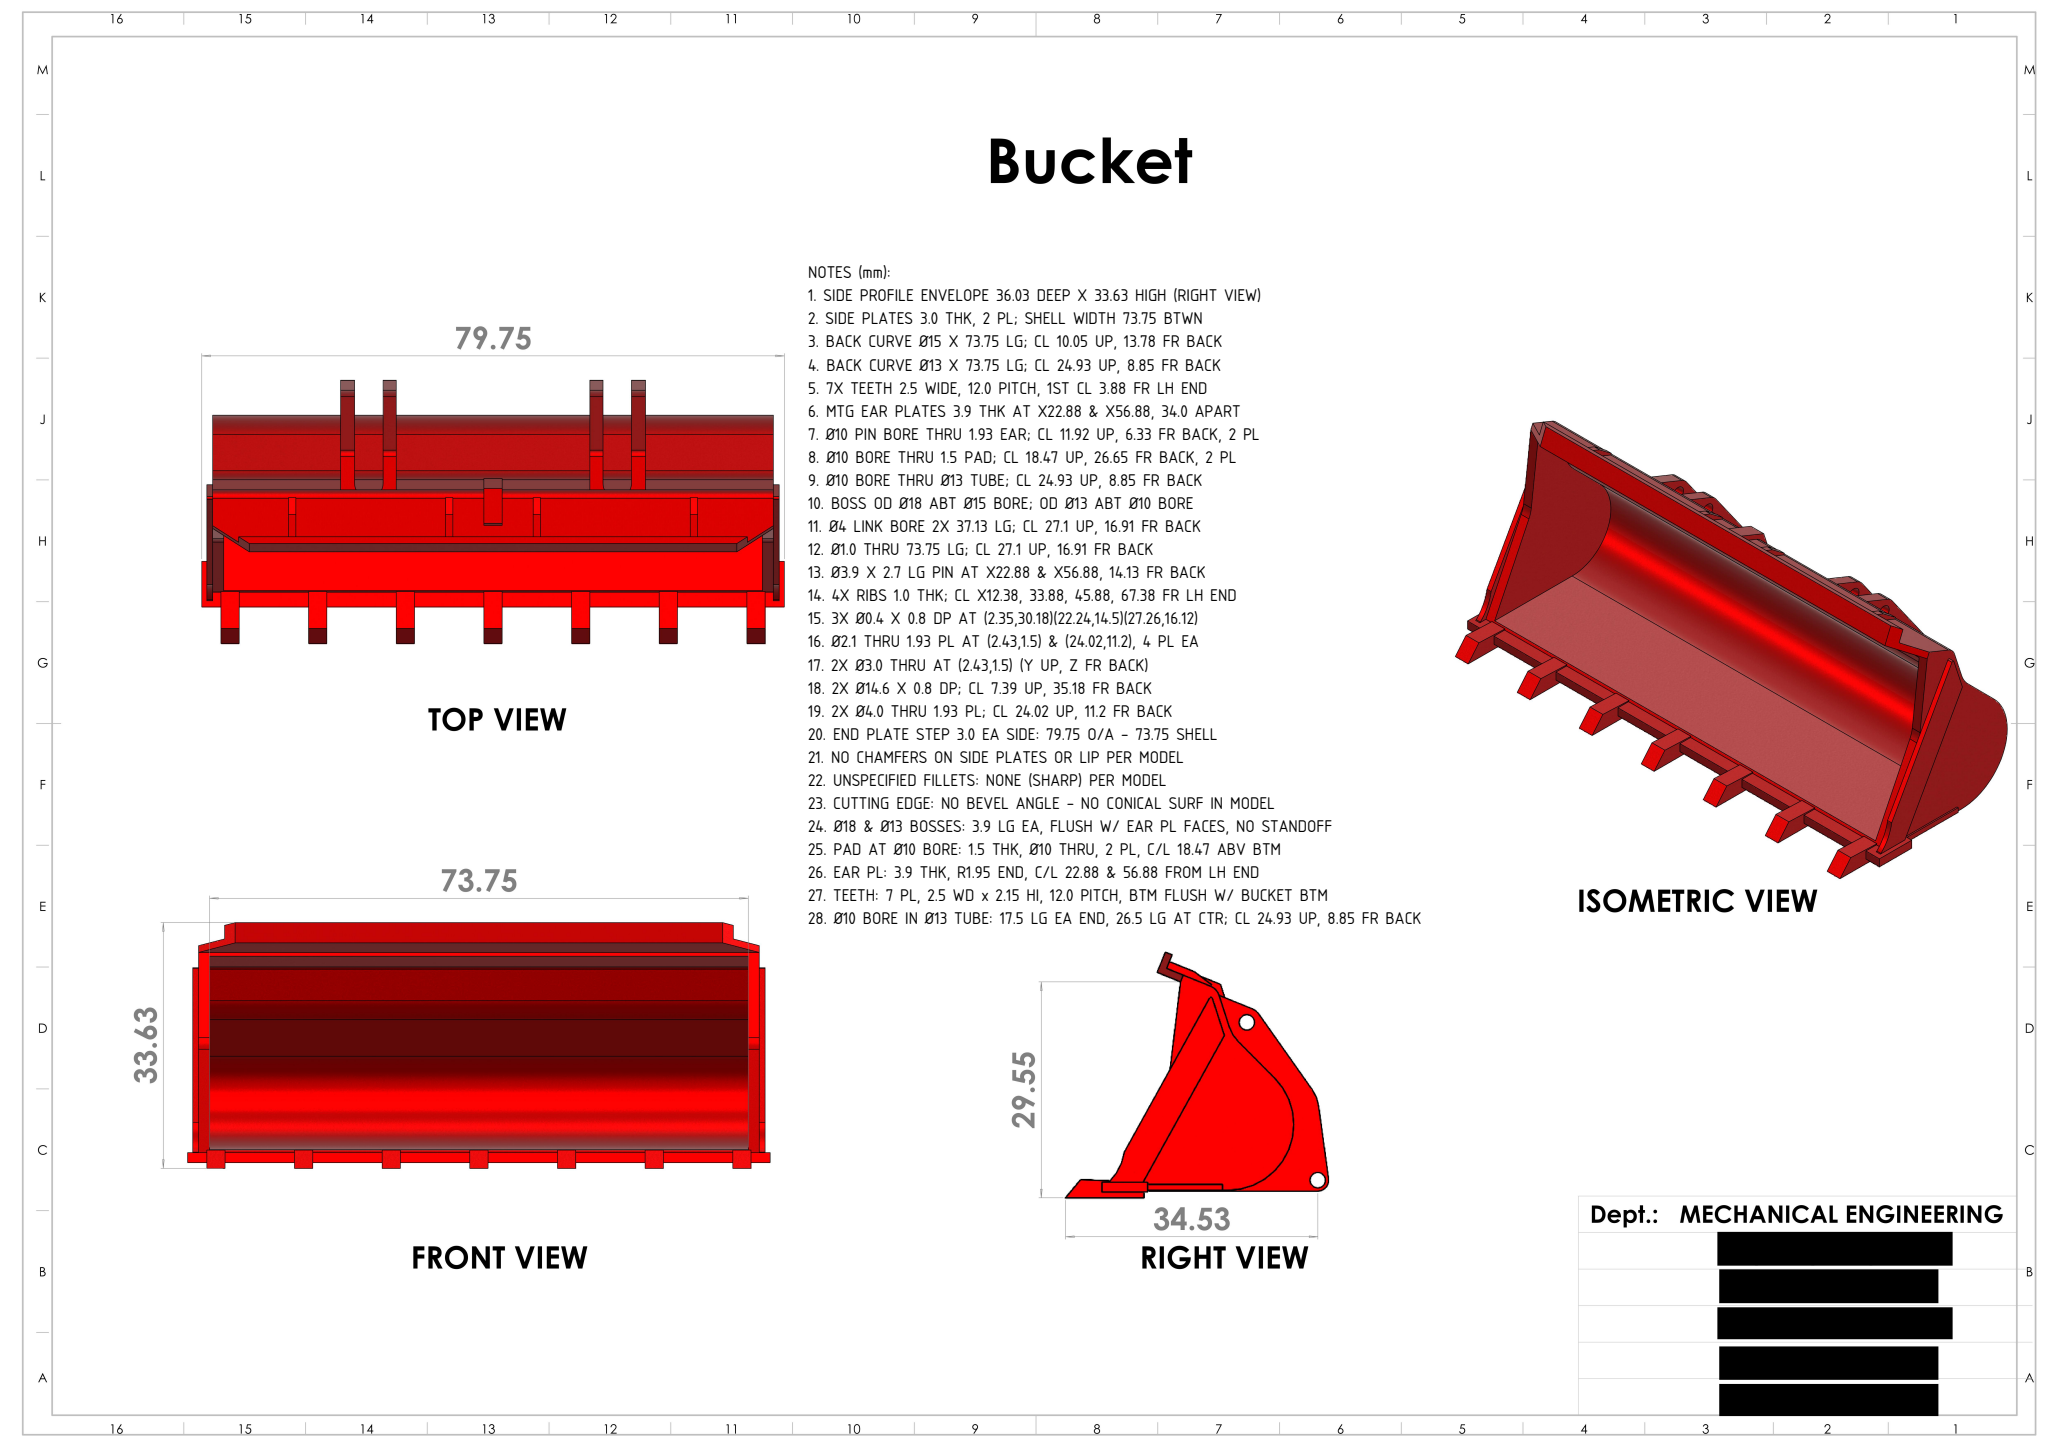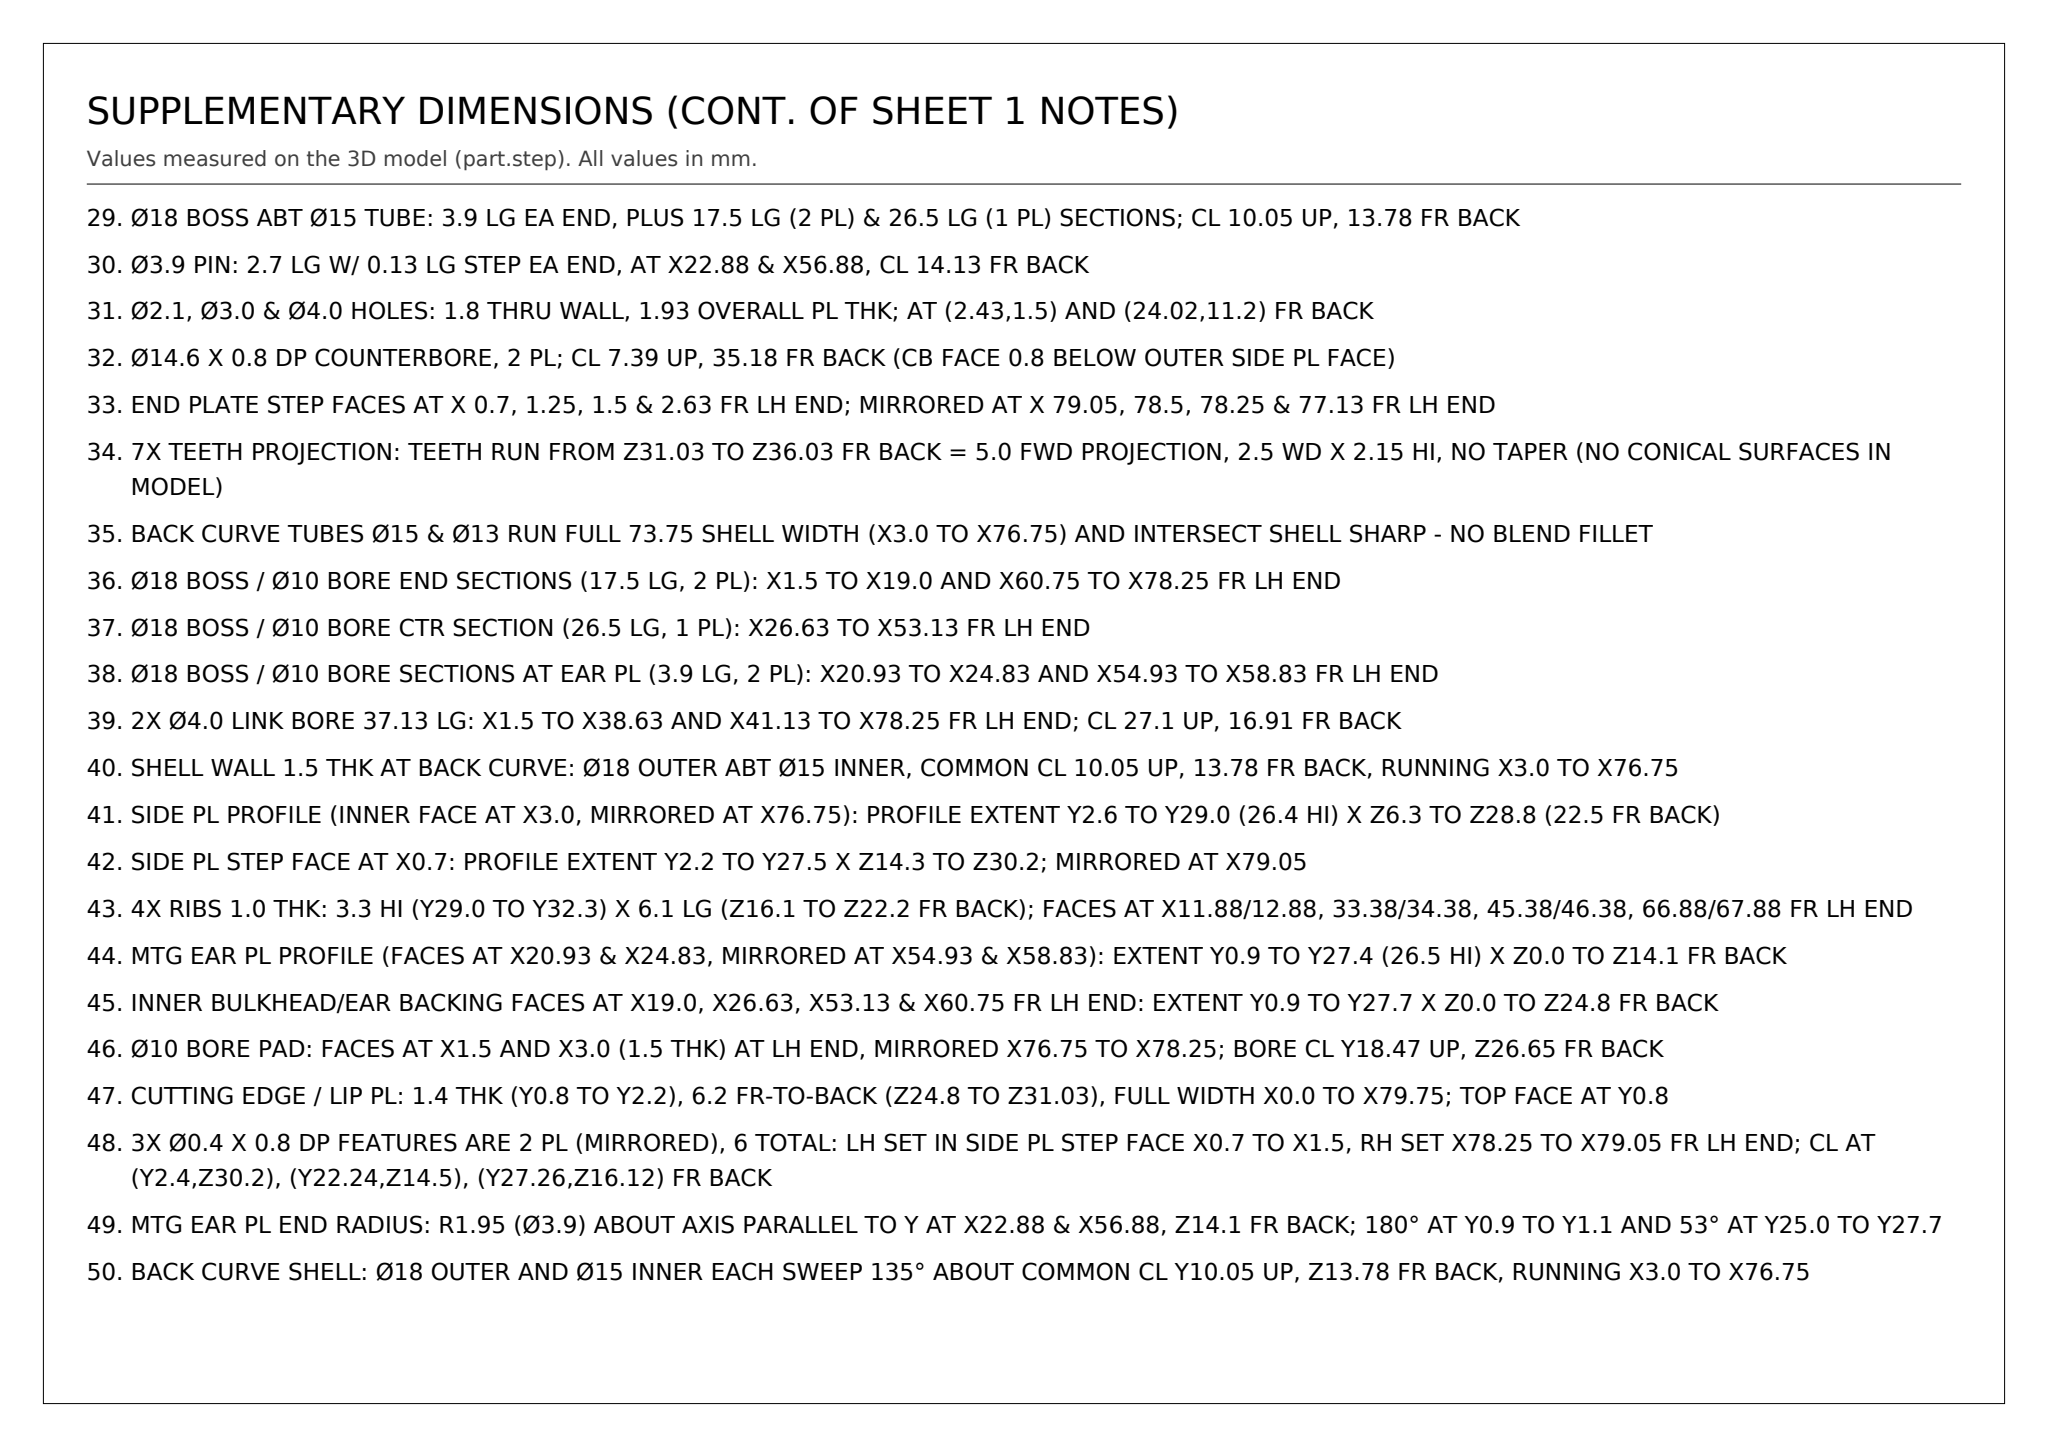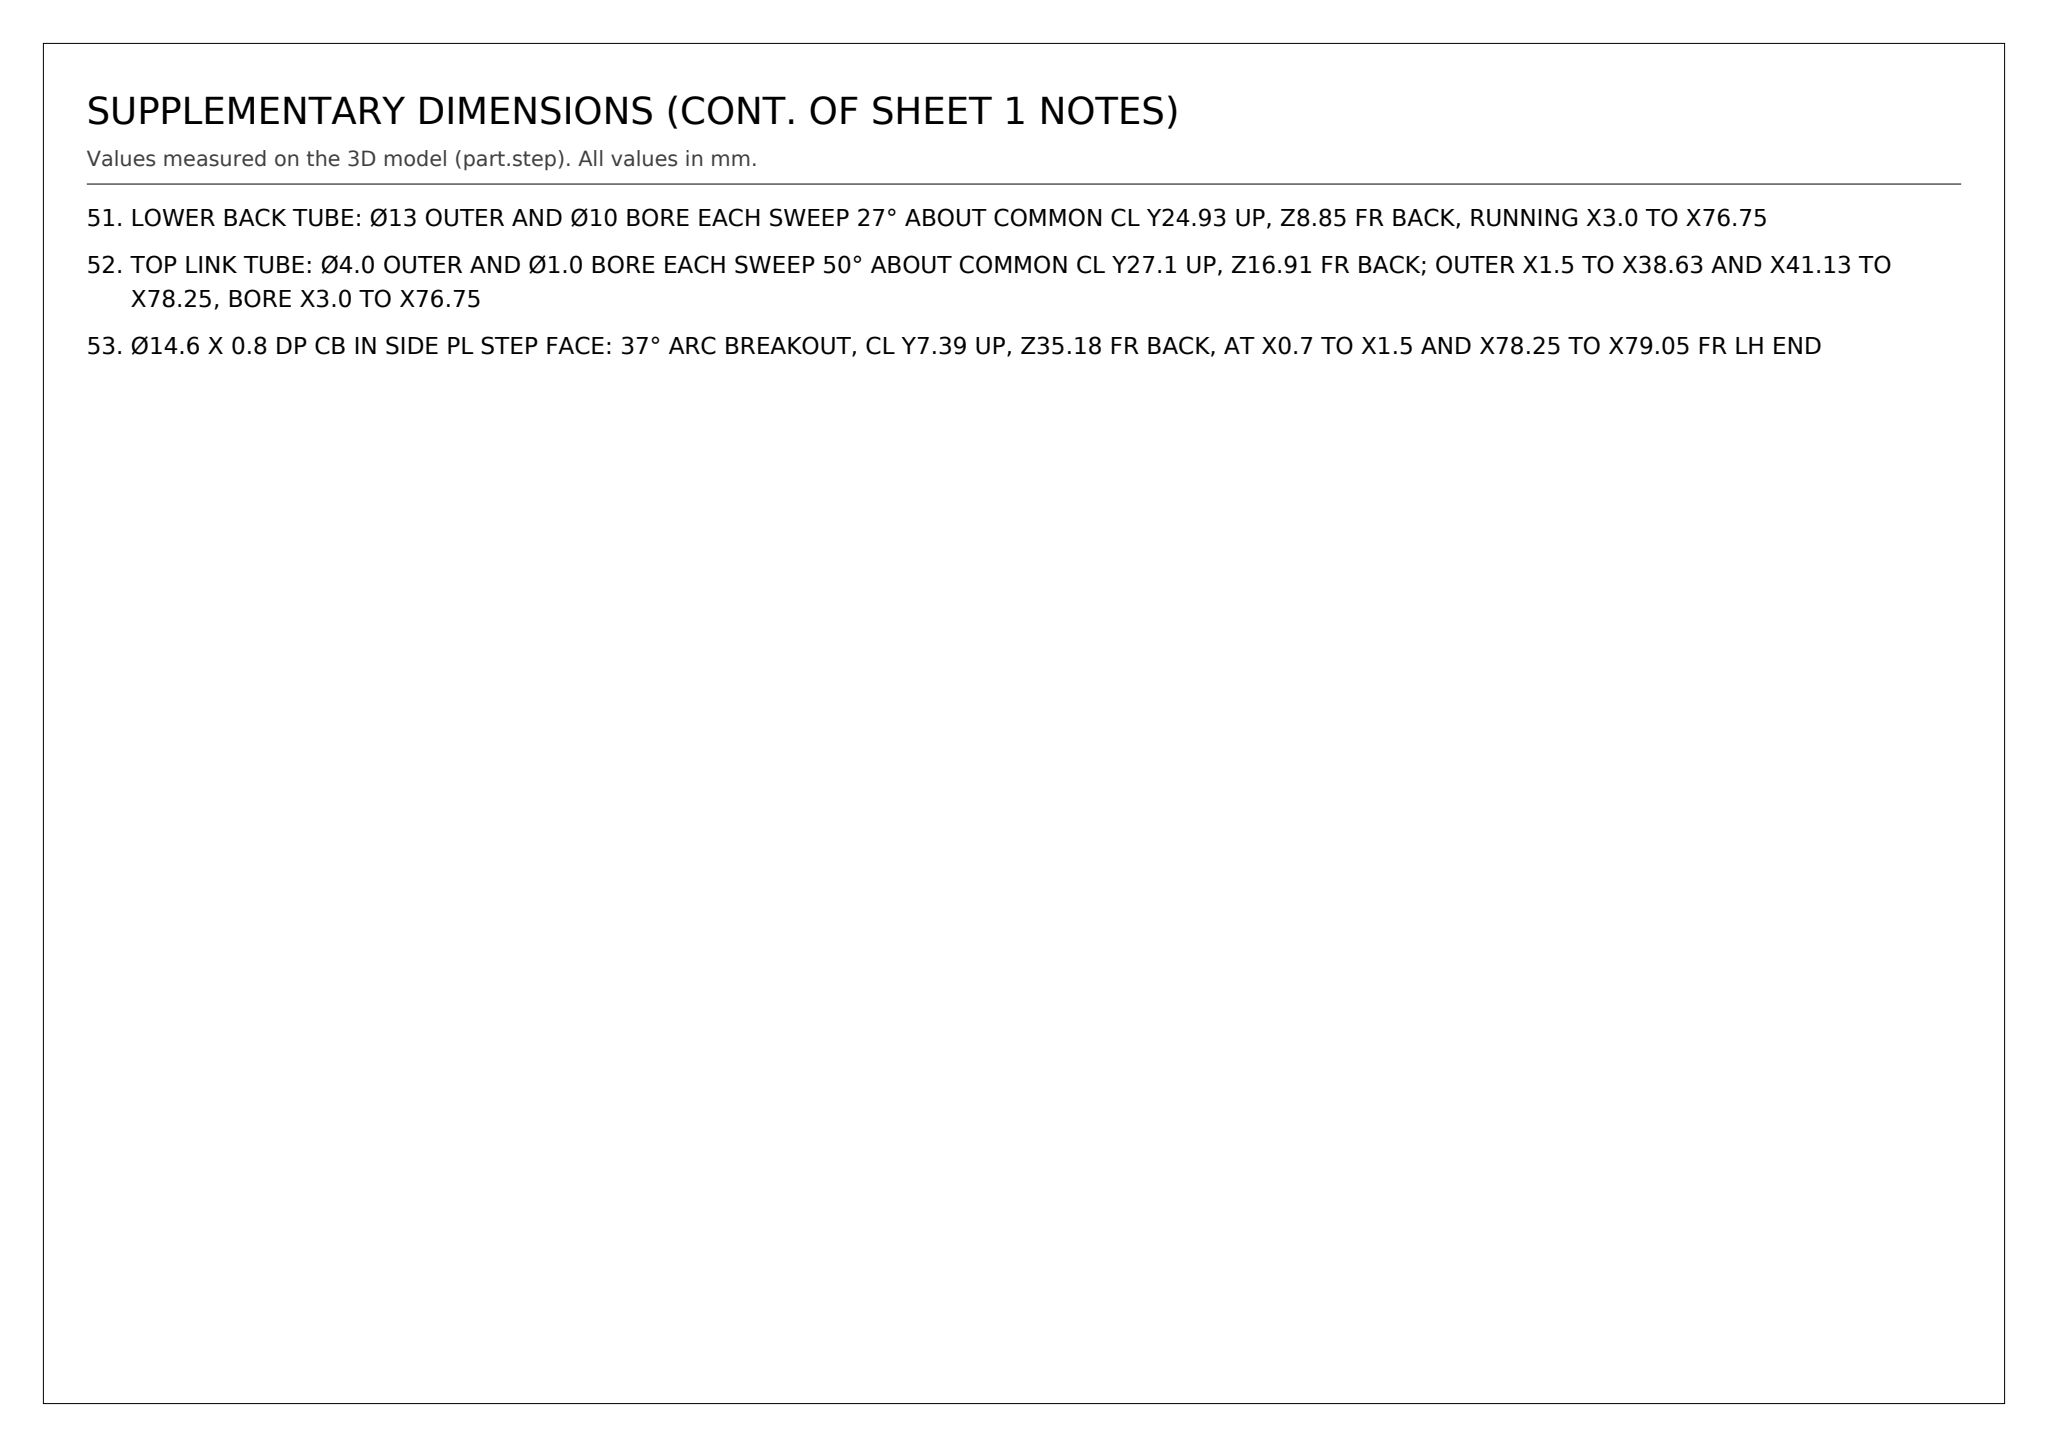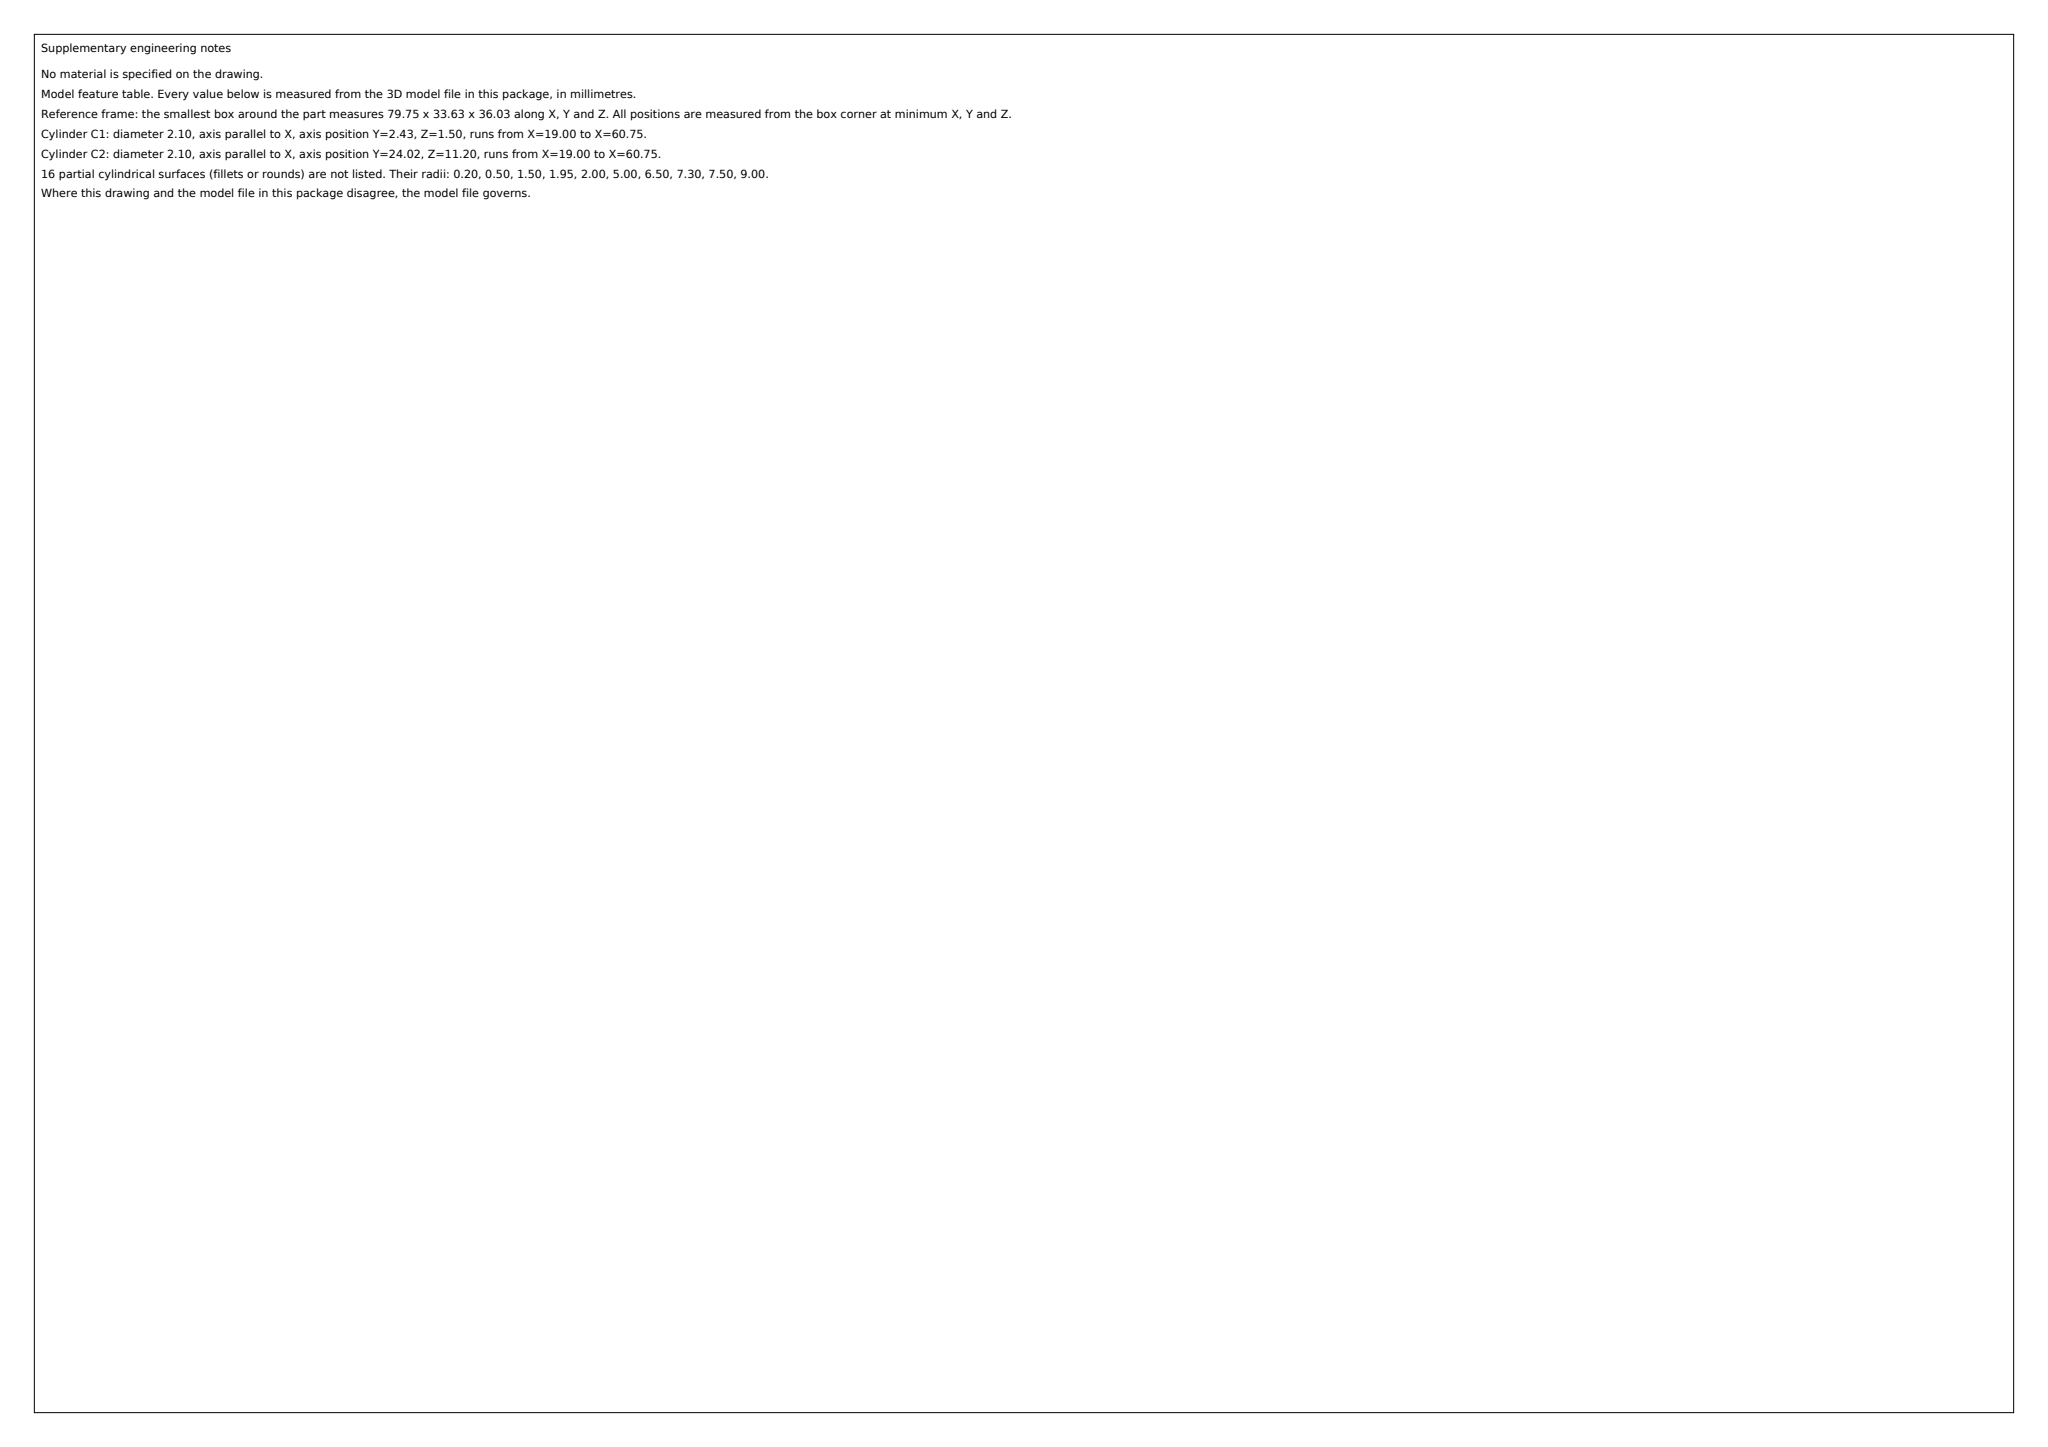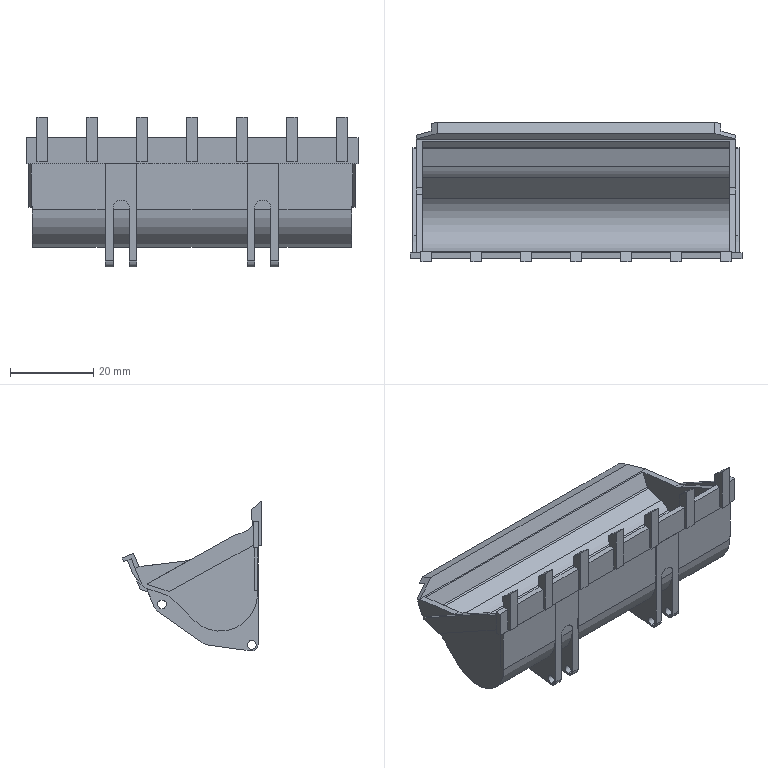Part | SolidWorks | mm | 1 solid | 223 faces | box 79.75 x 33.63 x 36.03 mm | volume 9342 mm3 | plane 162 | cylinder 61 | commonest cylinder face diameters 2.1 x16 10 x11 3.9 x8 4 x6 0.4 x6 18 x5 3 x4 14.6 x2
Drawing notes:
SIDE PROFILE ENVELOPE 36.03 DEEP X 33.63 HIGH (RIGHT VIEW) | from the solid: bbox_xyz = [79.75, 33.627, 36.031]
SIDE PLATES 3.0 THK, 2 PL; SHELL WIDTH 73.75 BTWN | from the solid: x planes 0.0/3.0 and 76.75/79.75; full-width cyls 73.75 lg
BACK CURVE Ø15 X 73.75 LG; CL 10.05 UP, 13.78 FR BACK | from the solid: [15,'x',[null,10.05,13.78],73.75,1]
BACK CURVE Ø13 X 73.75 LG; CL 24.93 UP, 8.85 FR BACK | from the solid: [13,'x',[null,24.93,8.85],73.75,1]
7X TEETH 2.5 WIDE, 12.0 PITCH, 1ST CL 3.88 FR LH END | from the solid: x planes 2.63/5.13, 14.63/17.13, 26.63/29.13, 38.63/41.13, 50.63/53.13, 62.63/65.13, 74.63/77.13
MTG EAR PLATES 3.9 THK AT X22.88 & X56.88, 34.0 APART | from the solid: x planes 20.93-24.83 & 54.93-58.83; Ø3.9 cyls at x=22.88 & 56.88
Ø10 PIN BORE THRU 1.93 EAR; CL 11.92 UP, 6.33 FR BACK, 2 PL | from the solid: [10,'x',[null,11.92,6.33],1.8,2] & [10,...,1.93,2]
Ø10 BORE THRU 1.5 PAD; CL 18.47 UP, 26.65 FR BACK, 2 PL | from the solid: [10,'x',[null,18.47,26.65],1.5,2]
Ø10 BORE THRU Ø13 TUBE; CL 24.93 UP, 8.85 FR BACK | from the solid: [10,'x',[null,24.93,8.85],3.9/17.5/26.5] coaxial w Ø13 x 73.75
BOSS OD Ø18 ABT Ø15 BORE; OD Ø13 ABT Ø10 BORE | from the solid: [18,'x',[null,10.05,13.78],3.9/17.5/26.5]; [13,'x',[null,24.93,8.85],73.75]
Ø4 LINK BORE 2X 37.13 LG; CL 27.1 UP, 16.91 FR BACK | from the solid: [4,'x',[null,27.1,16.91],37.13,2]
Ø1.0 THRU 73.75 LG; CL 27.1 UP, 16.91 FR BACK | from the solid: [1.0,'x',[null,27.1,16.91],73.75,1]
Ø3.9 X 2.7 LG PIN AT X22.88 & X56.88, 14.13 FR BACK | from the solid: [3.9,'y',[22.88,null,14.13],2.7,2] & [3.9,'y',[56.88,null,14.13],2.7,2]
4X RIBS 1.0 THK; CL X12.38, 33.88, 45.88, 67.38 FR LH END | from the solid: x plane pairs 11.88/12.88, 33.38/34.38, 45.38/46.38, 66.88/67.88
3X Ø0.4 X 0.8 DP AT (2.35,30.18)(22.24,14.5)(27.26,16.12) | from the solid: [0.4,'x',...,0.8,2] at y/z = 2.35/30.18, 22.24/14.5, 27.26/16.12
Ø2.1 THRU 1.93 PL AT (2.43,1.5) & (24.02,11.2), 4 PL EA | from the solid: [2.1,'x',[null,2.43,1.5],1.8/1.93,4]; [2.1,'x',[null,24.02,11.2],1.8/1.93,4]
2X Ø3.0 THRU AT (2.43,1.5) (Y UP, Z FR BACK) | from the solid: [3.0,'x',[null,2.43,1.5],1.8,2] & 1.93,2
2X Ø14.6 X 0.8 DP; CL 7.39 UP, 35.18 FR BACK | from the solid: [14.6,'x',[null,7.39,35.18],0.8,2]
2X Ø4.0 THRU 1.93 PL; CL 24.02 UP, 11.2 FR BACK | from the solid: [4.0,'x',[null,24.02,11.2],1.8,2] & 1.93,2
END PLATE STEP 3.0 EA SIDE: 79.75 O/A - 73.75 SHELL | from the solid: 79.75 bbox x vs 73.75 full-width cyls; x planes 3.0 & 76.75
NO CHAMFERS ON SIDE PLATES OR LIP PER MODEL | from the solid: cones[] empty in STEP data
UNSPECIFIED FILLETS: NONE (SHARP) PER MODEL | from the solid: fillet_radii[] empty in STEP data
CUTTING EDGE: NO BEVEL ANGLE - NO CONICAL SURF IN MODEL | from the solid: cones[included_angle,ref_dia] = []
Ø18 & Ø13 BOSSES: 3.9 LG EA, FLUSH W/ EAR PL FACES, NO STANDOFF | from the solid: Ø18 cyl L=3.9 (x2) @ y10.05/z13.78 and Ø10 cyl L=3.9 (x2) @ y24.93/z8.85 equal ear plate thk 3.9 (x planes 20.93-24.83 & 54.93-58.83)
PAD AT Ø10 BORE: 1.5 THK, Ø10 THRU, 2 PL, C/L 18.47 ABV BTM | from the solid: [10.0,'x',[null,18.47,26.65],1.5,2] - Ø10 bore, axial length 1.5 = pad thk, 2 places, C/L 18.47 from bbox min Y (bucket bottom)
EAR PL: 3.9 THK, R1.95 END, C/L 22.88 & 56.88 FROM LH END | from the solid: [3.9,'y',[22.88,null,14.13],2.7,2] & [3.9,'y',[56.88,null,14.13],...] rounded ends R1.95; x planes 20.93/24.83 & 54.93/58.83 = 3.9 thk, 34.0 apart
TEETH: 7 PL, 2.5 WD x 2.15 HI, 12.0 PITCH, BTM FLUSH W/ BUCKET BTM | from the solid: x plane pairs 2.63/5.13, 14.63/17.13, 26.63/29.13, 38.63/41.13, 50.63/53.13, 62.63/65.13, 74.63/77.13 = 2.5 wd @ 12.0 pitch; y=0 (7 faces) to y=2.15 (8 faces)
Ø10 BORE IN Ø13 TUBE: 17.5 LG EA END, 26.5 LG AT CTR; CL 24.93 UP, 8.85 FR BACK | from the solid: cylinders dia10 axis x at (24.93,8.85), lengths 17.5 (2 PL) and 26.5 (1 PL)
Ø18 BOSS ABT Ø15 TUBE: 3.9 LG EA END, PLUS 17.5 LG (2 PL) & 26.5 LG (1 PL) SECTIONS; CL 10.05 UP, 13.78 FR BACK | from the solid: cylinders dia18 axis x at (10.05,13.78), lengths 3.9 (2), 17.5 (2), 26.5 (1)
Ø3.9 PIN: 2.7 LG W/ 0.13 LG STEP EA END, AT X22.88 & X56.88, CL 14.13 FR BACK | from the solid: cylinders dia3.9 axis y at (22.88,14.13) and (56.88,14.13), lengths 2.7 and 0.13
Ø2.1, Ø3.0 & Ø4.0 HOLES: 1.8 THRU WALL, 1.93 OVERALL PL THK; AT (2.43,1.5) AND (24.02,11.2) FR BACK | from the solid: cylinders dia2.1/3.0/4.0 axis x at (2.43,1.5) & (24.02,11.2), lengths 1.8 and 1.93
Ø14.6 X 0.8 DP COUNTERBORE, 2 PL; CL 7.39 UP, 35.18 FR BACK (CB FACE 0.8 BELOW OUTER SIDE PL FACE) | from the solid: cylinders dia14.6 axis x at (7.39,35.18), length 0.8, count 2
END PLATE STEP FACES AT X 0.7, 1.25, 1.5 & 2.63 FR LH END; MIRRORED AT X 79.05, 78.5, 78.25 & 77.13 FR LH END | from the solid: axis_planes normal x at 0.7, 1.25, 1.5, 2.63 and 77.13, 78.25, 78.5, 79.05
7X TEETH PROJECTION: TEETH RUN FROM Z31.03 TO Z36.03 FR BACK = 5.0 FWD PROJECTION, 2.5 WD X 2.15 HI, NO TAPER (NO CONICAL SURFACES IN MODEL) | from the solid: axis_planes[z,31.03]:count 8 (tooth root faces) with bbox_xyz z = 36.031 front of envelope; cones[] empty
BACK CURVE TUBES Ø15 & Ø13 RUN FULL 73.75 SHELL WIDTH (X3.0 TO X76.75) AND INTERSECT SHELL SHARP - NO BLEND FILLET | from the solid: cylinders [15.0,x,(10.05,13.78),73.75] and [13.0,x,(24.93,8.85),73.75]; axis_planes x=3.0 and x=76.75; fillet_radii = [] (empty)
Ø18 BOSS / Ø10 BORE END SECTIONS (17.5 LG, 2 PL): X1.5 TO X19.0 AND X60.75 TO X78.25 FR LH END | from the solid: cylinders [18.0,x,(10.05,13.78),17.5,2] and [10.0,x,(24.93,8.85),17.5,2]; x planes 1.5, 19.0, 60.75, 78.25
Ø18 BOSS / Ø10 BORE CTR SECTION (26.5 LG, 1 PL): X26.63 TO X53.13 FR LH END | from the solid: cylinders [18.0,x,(10.05,13.78),26.5,1] and [10.0,x,(24.93,8.85),26.5,1]; x planes 26.63, 53.13
Ø18 BOSS / Ø10 BORE SECTIONS AT EAR PL (3.9 LG, 2 PL): X20.93 TO X24.83 AND X54.93 TO X58.83 FR LH END | from the solid: cylinders [18.0,x,(10.05,13.78),3.9,2] and [10.0,x,(24.93,8.85),3.9,2]; x planes 20.93, 24.83, 54.93, 58.83
2X Ø4.0 LINK BORE 37.13 LG: X1.5 TO X38.63 AND X41.13 TO X78.25 FR LH END; CL 27.1 UP, 16.91 FR BACK | from the solid: cylinder [4.0,x,(27.1,16.91),37.13,2]; x planes 1.5, 38.63, 41.13, 78.25
SHELL WALL 1.5 THK AT BACK CURVE: Ø18 OUTER ABT Ø15 INNER, COMMON CL 10.05 UP, 13.78 FR BACK, RUNNING X3.0 TO X76.75 | from the solid: concave arc Ø15 x-axis at (y10.1,z13.8) x3.0-76.8 and convex arc Ø18 x-axis at same (y10.1,z13.8) spanning x1.5-78.25 (coaxial, radial difference 1.5)
SIDE PL PROFILE (INNER FACE AT X3.0, MIRRORED AT X76.75): PROFILE EXTENT Y2.6 TO Y29.0 (26.4 HI) X Z6.3 TO Z28.8 (22.5 FR BACK) | from the solid: axis_plane x=3.0 extent y[2.6,29.0] z[6.3,28.8] area 331 (and mirror x=76.8 same extent)
SIDE PL STEP FACE AT X0.7: PROFILE EXTENT Y2.2 TO Y27.5 X Z14.3 TO Z30.2; MIRRORED AT X79.05 | from the solid: axis_plane x=0.7 extent y[2.2,27.5] z[14.3,30.2] area 109 (mirror x=79.1)
4X RIBS 1.0 THK: 3.3 HI (Y29.0 TO Y32.3) X 6.1 LG (Z16.1 TO Z22.2 FR BACK); FACES AT X11.88/12.88, 33.38/34.38, 45.38/46.38, 66.88/67.88 FR LH END | from the solid: axis_planes x=11.9,12.9,33.4,34.4,45.4,46.4,66.9,67.9 each extent y[29.0,32.3] z[16.1,22.2] area 5
MTG EAR PL PROFILE (FACES AT X20.93 & X24.83, MIRRORED AT X54.93 & X58.83): EXTENT Y0.9 TO Y27.4 (26.5 HI) X Z0.0 TO Z14.1 FR BACK | from the solid: axis_planes x=20.9, 24.8, 54.9, 58.8 each extent y[0.9,27.4] z[0.0,14.1] area 124
INNER BULKHEAD/EAR BACKING FACES AT X19.0, X26.63, X53.13 & X60.75 FR LH END: EXTENT Y0.9 TO Y27.7 X Z0.0 TO Z24.8 FR BACK | from the solid: axis_planes x=19.0, 26.6, 53.1, 60.8 each extent y[0.9,27.7] z[0.0,24.8] area 127
Ø10 BORE PAD: FACES AT X1.5 AND X3.0 (1.5 THK) AT LH END, MIRRORED X76.75 TO X78.25; BORE CL Y18.47 UP, Z26.65 FR BACK | from the solid: concave arc Ø10 x-axis at (y18.5,z26.6) from x1.5 to 3.0 and from x76.8 to 78.3
CUTTING EDGE / LIP PL: 1.4 THK (Y0.8 TO Y2.2), 6.2 FR-TO-BACK (Z24.8 TO Z31.03), FULL WIDTH X0.0 TO X79.75; TOP FACE AT Y0.8 | from the solid: axis_plane y=0.8 extent x[0.0,79.8] z[24.8,31.0] area 398; axis_plane x=0.0 extent y[0.8,2.2] z[24.8,31.0] area 8
3X Ø0.4 X 0.8 DP FEATURES ARE 2 PL (MIRRORED), 6 TOTAL: LH SET IN SIDE PL STEP FACE X0.7 TO X1.5, RH SET X78.25 TO X79.05 FR LH END; CL AT (Y2.4,Z30.2), (Y22.24,Z14.5), (Y27.26,Z16.12) FR BACK | from the solid: cylinders dia 0.4 about x-axis at (y2.4,z30.2), (y22.2,z14.5), (y27.3,z16.1), each present from x0.7-1.5 and from x78.2-79.1
MTG EAR PL END RADIUS: R1.95 (Ø3.9) ABOUT AXIS PARALLEL TO Y AT X22.88 & X56.88, Z14.1 FR BACK; 180° AT Y0.9 TO Y1.1 AND 53° AT Y25.0 TO Y27.7 | from the solid: concave arcs dia 3.9, axis y, at (x22.9,z14.1) and (x56.9,z14.1), from y0.9-1.1 arc 180 deg and from y25.0-27.7 arc 53 deg
BACK CURVE SHELL: Ø18 OUTER AND Ø15 INNER EACH SWEEP 135° ABOUT COMMON CL Y10.05 UP, Z13.78 FR BACK, RUNNING X3.0 TO X76.75 | from the solid: convex arc dia 18 and concave arc dia 15 about x-axis at (y10.1,z13.8), x3.0 to 76.8, arc_deg 135
LOWER BACK TUBE: Ø13 OUTER AND Ø10 BORE EACH SWEEP 27° ABOUT COMMON CL Y24.93 UP, Z8.85 FR BACK, RUNNING X3.0 TO X76.75 | from the solid: convex arc dia 13 (x3.0-76.8) and concave arc dia 10 at (y24.9,z8.9), arc_deg 27
TOP LINK TUBE: Ø4.0 OUTER AND Ø1.0 BORE EACH SWEEP 50° ABOUT COMMON CL Y27.1 UP, Z16.91 FR BACK; OUTER X1.5 TO X38.63 AND X41.13 TO X78.25, BORE X3.0 TO X76.75 | from the solid: convex arc dia 4.0 about x at (y27.1,z16.9) from x1.5-38.6 and x41.1-78.3, arc 50 deg; concave arc dia 1.0 same CL x3.0-76.8, arc 50 deg
Ø14.6 X 0.8 DP CB IN SIDE PL STEP FACE: 37° ARC BREAKOUT, CL Y7.39 UP, Z35.18 FR BACK, AT X0.7 TO X1.5 AND X78.25 TO X79.05 FR LH END | from the solid: concave arc dia 14.6 about x at (y7.4,z35.2), from x0.7-1.5 and x78.2-79.1, arc_deg 37